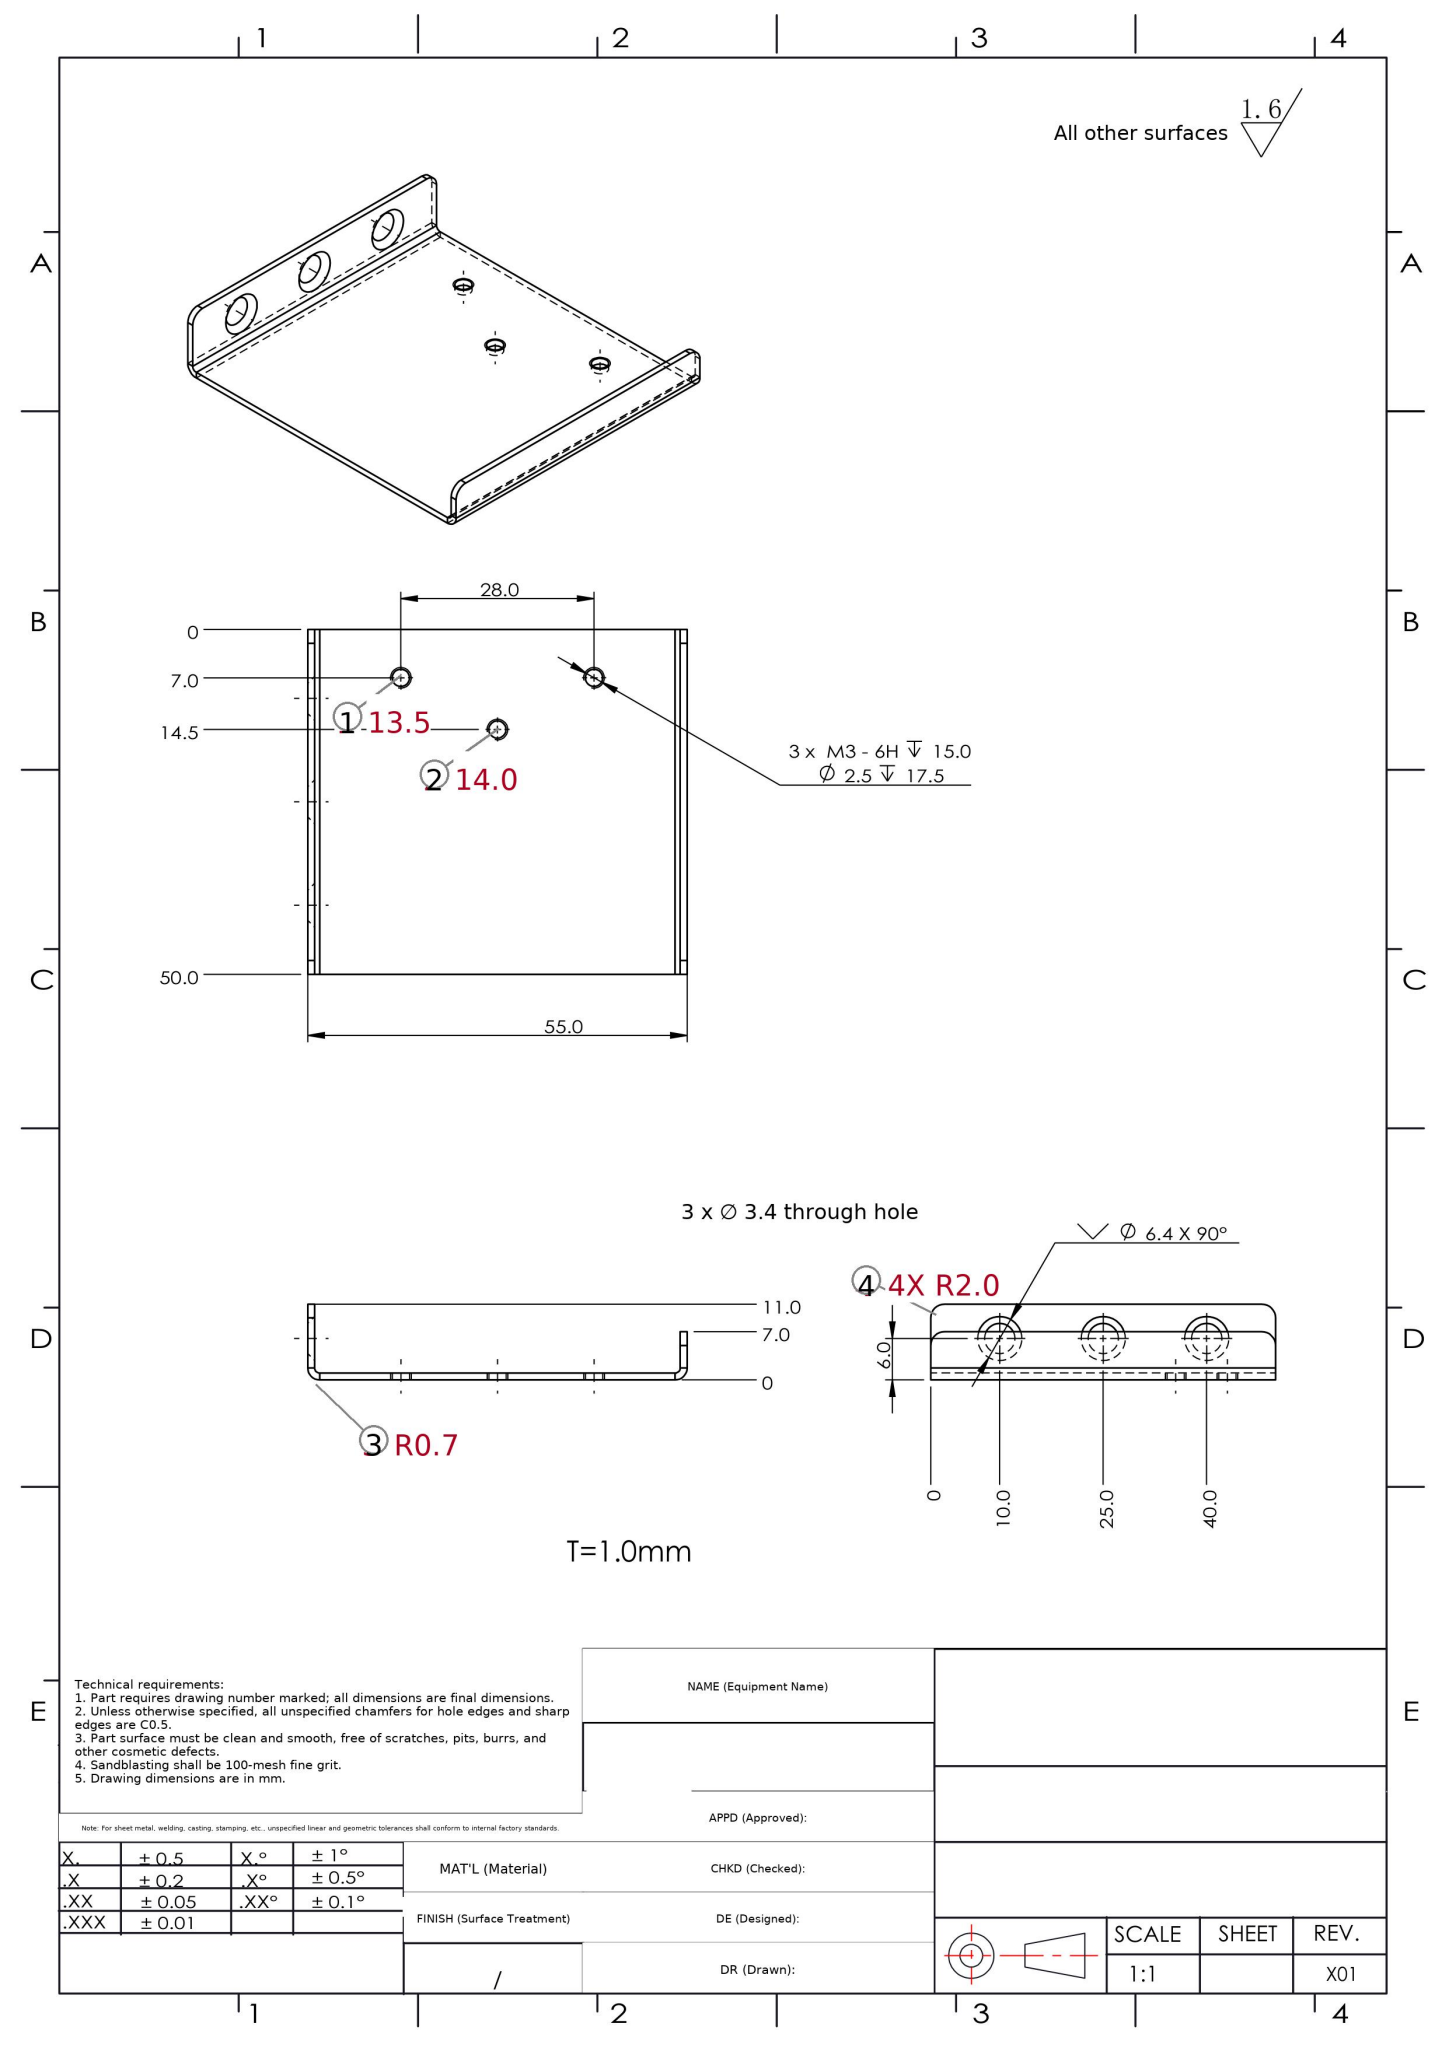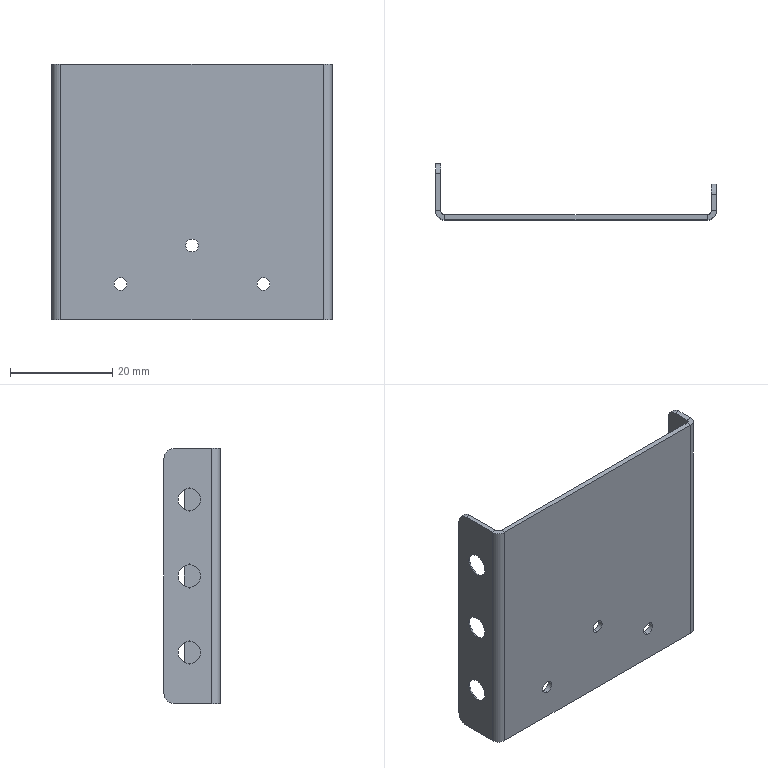Part | SolidWorks | mm | 1 solid | 38 faces | box 55 x 11 x 50 mm | volume 3409 mm3 | plane 18 | cylinder 14 | cone 6 | commonest cylinder face diameters 2.5 x6 4 x4 1.473 x2 3.473 x2